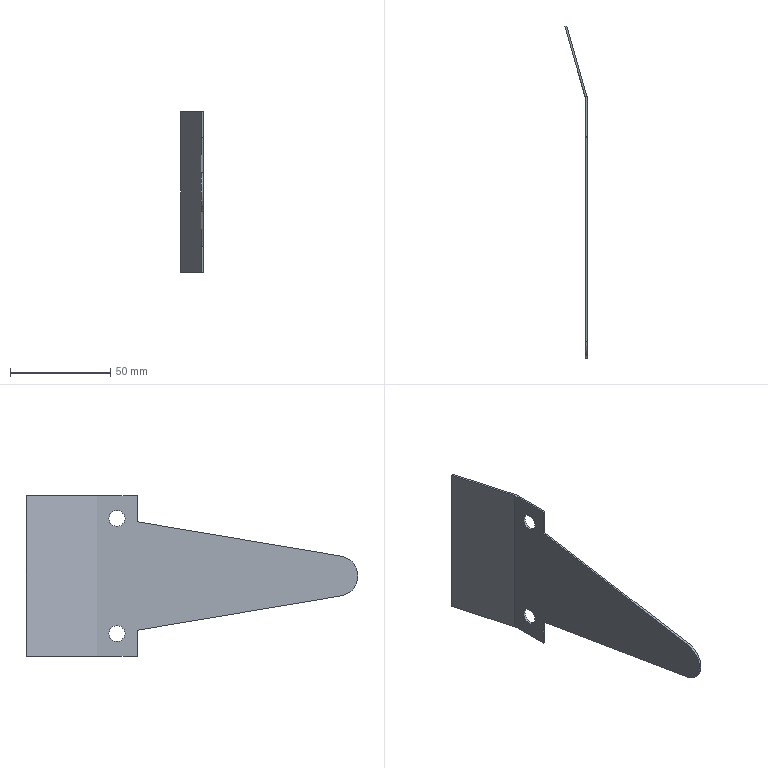Component | SolidWorks | OuterBagExpansionSheetMetal-1 | 2 solids | 21 faces | box 11.04 x 165.28 x 80 mm | volume 8295 mm3 | plane 15 | cylinder 6 | commonest cylinder face diameters 8 x4 2 x1 20 x1
build123d program:
from build123d import *

# Parameters (mm, degrees)
BOSS_EXTRUDE1_DEPTH = 1
SKETCH3_R           = 4
CUT_EXTRUDE1_DEPTH  = 10
BOSS_EXTRUDE2_DEPTH = 80


with BuildPart() as part:
    # Sketch2 → Boss-Extrude1 (new body)
    with BuildSketch(Plane.XY):
        with BuildLine():
            Line((0.831, 140.622), (102.493, 157.762))
            ThreePointArc((102.493, 157.762), (110.831, 167.622), (102.493, 177.483))
            Line((102.493, 177.483), (0.831, 194.622))
            Line((0.831, 194.622), (0.831, 207.622))
            Line((0.831, 207.622), (-19.169, 207.622))
            Line((-19.169, 207.622), (-19.169, 127.622))
            Line((-19.169, 127.622), (0.831, 127.622))
            Line((0.831, 127.622), (0.831, 140.622))
        make_face()
    extrude(amount=BOSS_EXTRUDE1_DEPTH)

    # Sketch3 → Cut-Extrude1 (cut)
    with BuildSketch(Plane.XY.offset(1)):
        with Locations((-9.169, 138.937)):
            Circle(SKETCH3_R)
        with Locations((-9.169, 196.308)):
            Circle(SKETCH3_R)
    extrude(amount=-CUT_EXTRUDE1_DEPTH, mode=Mode.SUBTRACT)


with BuildPart() as body_2:
    # Sketch4 → Boss-Extrude2 (new body)
    with BuildSketch(Plane(origin=(0, 207.622, 0), x_dir=(1, 0, 0), z_dir=(0, 1, 0))):
        with BuildLine():
            Line((-19.169, -1), (-19.169, 0))
            Line((-19.169, 0), (-54.169, 10.036))
            Line((-54.169, 10.036), (-54.445, 9.075))
            Line((-54.445, 9.075), (-19.445, -0.9613))
            ThreePointArc((-19.445, -0.9613), (-19.308, -0.9903), (-19.169, -1))
        make_face()
    extrude(amount=-BOSS_EXTRUDE2_DEPTH)


solid = Compound([part.part, body_2.part])

# Placed as in the assembly
solid = solid.moved(Location((-550.446, 3.257, 541.09), (-90, 90, 0)))
STEP:
#1=COLOUR_RGB('',0.7922,0.8196,0.9333);
#2=FILL_AREA_STYLE_COLOUR('',#1);
#3=FILL_AREA_STYLE('',(#2));
#4=SURFACE_STYLE_FILL_AREA(#3);
#5=SURFACE_SIDE_STYLE('',(#4));
#6=SURFACE_STYLE_USAGE(.BOTH.,#5);
#7=PRESENTATION_STYLE_ASSIGNMENT((#6));
#8=CARTESIAN_POINT('',(-21.633,0.8938,13.129));
#9=VERTEX_POINT('',#8);
#10=CARTESIAN_POINT('',(-21.632,0.8829,13.129));
#11=VERTEX_POINT('',#10);
#12=CARTESIAN_POINT('',(-21.671,0.8829,13.129));
#13=DIRECTION('',(0.,0.,-1.));
#14=DIRECTION('',(1.,0.,0.));
#15=AXIS2_PLACEMENT_3D('',#12,#13,#14);
#16=CIRCLE('',#15,0.03937);
#17=EDGE_CURVE('',#9,#11,#16,.T.);
#18=ORIENTED_EDGE('',*,*,#17,.F.);
#19=CARTESIAN_POINT('',(-21.633,0.8938,16.278));
#20=VERTEX_POINT('',#19);
#21=CARTESIAN_POINT('',(-21.633,0.8938,16.278));
#22=DIRECTION('',(0.,0.,-1.));
#23=VECTOR('',#22,39.37);
#24=LINE('',#21,#23);
#25=EDGE_CURVE('',#20,#9,#24,.T.);
#26=ORIENTED_EDGE('',*,*,#25,.F.);
#27=CARTESIAN_POINT('',(-21.632,0.8829,16.278));
#28=VERTEX_POINT('',#27);
#29=CARTESIAN_POINT('',(-21.671,0.8829,16.278));
#30=DIRECTION('',(0.,0.,-1.));
#31=DIRECTION('',(1.,0.,0.));
#32=AXIS2_PLACEMENT_3D('',#29,#30,#31);
#33=CIRCLE('',#32,0.03937);
#34=EDGE_CURVE('',#20,#28,#33,.T.);
#35=ORIENTED_EDGE('',*,*,#34,.T.);
#36=CARTESIAN_POINT('',(-21.632,0.8829,16.278));
#37=DIRECTION('',(0.,0.,-1.));
#38=VECTOR('',#37,39.37);
#39=LINE('',#36,#38);
#40=EDGE_CURVE('',#28,#11,#39,.T.);
#41=ORIENTED_EDGE('',*,*,#40,.T.);
#42=EDGE_LOOP('',(#18,#26,#35,#41));
#43=FACE_OUTER_BOUND('',#42,.T.);
#44=CARTESIAN_POINT('',(-21.671,0.8829,16.278));
#45=DIRECTION('',(0.,0.,-1.));
#46=DIRECTION('',(1.,0.,0.));
#47=AXIS2_PLACEMENT_3D('',#44,#45,#46);
#48=CYLINDRICAL_SURFACE('',#47,0.03937);
#49=ADVANCED_FACE('',(#43),#48,.T.);
#50=CARTESIAN_POINT('',(-22.028,2.272,13.129));
#51=VERTEX_POINT('',#50);
#52=CARTESIAN_POINT('',(-21.633,0.8938,13.129));
#53=DIRECTION('',(0.2756,-0.9613,-0.));
#54=VECTOR('',#53,39.37);
#55=LINE('',#52,#54);
#56=EDGE_CURVE('',#51,#9,#55,.T.);
#57=ORIENTED_EDGE('',*,*,#56,.F.);
#58=CARTESIAN_POINT('',(-22.028,2.272,16.278));
#59=VERTEX_POINT('',#58);
#60=CARTESIAN_POINT('',(-22.028,2.272,16.278));
#61=DIRECTION('',(0.,0.,-1.));
#62=VECTOR('',#61,39.37);
#63=LINE('',#60,#62);
#64=EDGE_CURVE('',#59,#51,#63,.T.);
#65=ORIENTED_EDGE('',*,*,#64,.F.);
#66=CARTESIAN_POINT('',(-21.633,0.8938,16.278));
#67=DIRECTION('',(0.2756,-0.9613,-0.));
#68=VECTOR('',#67,39.37);
#69=LINE('',#66,#68);
#70=EDGE_CURVE('',#59,#20,#69,.T.);
#71=ORIENTED_EDGE('',*,*,#70,.T.);
#72=ORIENTED_EDGE('',*,*,#25,.T.);
#73=EDGE_LOOP('',(#57,#65,#71,#72));
#74=FACE_OUTER_BOUND('',#73,.T.);
#75=CARTESIAN_POINT('',(-21.633,0.8938,16.278));
#76=DIRECTION('',(0.9613,0.2756,0.));
#77=DIRECTION('',(0.2756,-0.9613,-0.));
#78=AXIS2_PLACEMENT_3D('',#75,#76,#77);
#79=PLANE('',#78);
#80=ADVANCED_FACE('',(#74),#79,.T.);
#81=CARTESIAN_POINT('',(-22.066,2.261,13.129));
#82=VERTEX_POINT('',#81);
#83=CARTESIAN_POINT('',(-22.066,2.261,13.129));
#84=DIRECTION('',(0.9613,0.2756,0.));
#85=VECTOR('',#84,39.37);
#86=LINE('',#83,#85);
#87=EDGE_CURVE('',#82,#51,#86,.T.);
#88=ORIENTED_EDGE('',*,*,#87,.F.);
#89=CARTESIAN_POINT('',(-22.066,2.261,16.278));
#90=VERTEX_POINT('',#89);
#91=CARTESIAN_POINT('',(-22.066,2.261,16.278));
#92=DIRECTION('',(0.,0.,-1.));
#93=VECTOR('',#92,39.37);
#94=LINE('',#91,#93);
#95=EDGE_CURVE('',#90,#82,#94,.T.);
#96=ORIENTED_EDGE('',*,*,#95,.F.);
#97=CARTESIAN_POINT('',(-22.066,2.261,16.278));
#98=DIRECTION('',(0.9613,0.2756,0.));
#99=VECTOR('',#98,39.37);
#100=LINE('',#97,#99);
#101=EDGE_CURVE('',#90,#59,#100,.T.);
#102=ORIENTED_EDGE('',*,*,#101,.T.);
#103=ORIENTED_EDGE('',*,*,#64,.T.);
#104=EDGE_LOOP('',(#88,#96,#102,#103));
#105=FACE_OUTER_BOUND('',#104,.T.);
#106=CARTESIAN_POINT('',(-22.066,2.261,16.278));
#107=DIRECTION('',(-0.2756,0.9613,0.));
#108=DIRECTION('',(0.9613,0.2756,0.));
#109=AXIS2_PLACEMENT_3D('',#106,#107,#108);
#110=PLANE('',#109);
#111=ADVANCED_FACE('',(#105),#110,.T.);
#112=CARTESIAN_POINT('',(-21.671,0.8829,13.129));
#113=VERTEX_POINT('',#112);
#114=CARTESIAN_POINT('',(-21.671,0.8829,13.129));
#115=DIRECTION('',(-0.2756,0.9613,0.));
#116=VECTOR('',#115,39.37);
#117=LINE('',#114,#116);
#118=EDGE_CURVE('',#113,#82,#117,.T.);
#119=ORIENTED_EDGE('',*,*,#118,.F.);
#120=CARTESIAN_POINT('',(-21.671,0.8829,16.278));
#121=VERTEX_POINT('',#120);
#122=CARTESIAN_POINT('',(-21.671,0.8829,16.278));
#123=DIRECTION('',(0.,0.,-1.));
#124=VECTOR('',#123,39.37);
#125=LINE('',#122,#124);
#126=EDGE_CURVE('',#121,#113,#125,.T.);
#127=ORIENTED_EDGE('',*,*,#126,.F.);
#128=CARTESIAN_POINT('',(-21.671,0.8829,16.278));
#129=DIRECTION('',(-0.2756,0.9613,0.));
#130=VECTOR('',#129,39.37);
#131=LINE('',#128,#130);
#132=EDGE_CURVE('',#121,#90,#131,.T.);
#133=ORIENTED_EDGE('',*,*,#132,.T.);
#134=ORIENTED_EDGE('',*,*,#95,.T.);
#135=EDGE_LOOP('',(#119,#127,#133,#134));
#136=FACE_OUTER_BOUND('',#135,.T.);
#137=CARTESIAN_POINT('',(-21.671,0.8829,16.278));
#138=DIRECTION('',(-0.9613,-0.2756,-0.));
#139=DIRECTION('',(-0.2756,0.9613,0.));
#140=AXIS2_PLACEMENT_3D('',#137,#138,#139);
#141=PLANE('',#140);
#142=ADVANCED_FACE('',(#136),#141,.T.);
#143=CARTESIAN_POINT('',(-21.632,0.8829,13.129));
#144=DIRECTION('',(-1.,0.,-0.));
#145=VECTOR('',#144,39.37);
#146=LINE('',#143,#145);
#147=EDGE_CURVE('',#11,#113,#146,.T.);
#148=ORIENTED_EDGE('',*,*,#147,.F.);
#149=ORIENTED_EDGE('',*,*,#40,.F.);
#150=CARTESIAN_POINT('',(-21.632,0.8829,16.278));
#151=DIRECTION('',(-1.,0.,-0.));
#152=VECTOR('',#151,39.37);
#153=LINE('',#150,#152);
#154=EDGE_CURVE('',#28,#121,#153,.T.);
#155=ORIENTED_EDGE('',*,*,#154,.T.);
#156=ORIENTED_EDGE('',*,*,#126,.T.);
#157=EDGE_LOOP('',(#148,#149,#155,#156));
#158=FACE_OUTER_BOUND('',#157,.T.);
#159=CARTESIAN_POINT('',(-21.632,0.8829,16.278));
#160=DIRECTION('',(-0.,-1.,-0.));
#161=DIRECTION('',(-1.,0.,-0.));
#162=AXIS2_PLACEMENT_3D('',#159,#160,#161);
#163=PLANE('',#162);
#164=ADVANCED_FACE('',(#158),#163,.T.);
#165=ORIENTED_EDGE('',*,*,#34,.F.);
#166=ORIENTED_EDGE('',*,*,#70,.F.);
#167=ORIENTED_EDGE('',*,*,#101,.F.);
#168=ORIENTED_EDGE('',*,*,#132,.F.);
#169=ORIENTED_EDGE('',*,*,#154,.F.);
#170=EDGE_LOOP('',(#165,#166,#167,#168,#169));
#171=FACE_OUTER_BOUND('',#170,.T.);
#172=CARTESIAN_POINT('',(-21.671,0.8829,16.278));
#173=DIRECTION('',(0.,0.,-1.));
#174=DIRECTION('',(1.,-0.,0.));
#175=AXIS2_PLACEMENT_3D('',#172,#173,#174);
#176=PLANE('',#175);
#177=ADVANCED_FACE('',(#171),#176,.F.);
#178=ORIENTED_EDGE('',*,*,#17,.T.);
#179=ORIENTED_EDGE('',*,*,#147,.T.);
#180=ORIENTED_EDGE('',*,*,#118,.T.);
#181=ORIENTED_EDGE('',*,*,#87,.T.);
#182=ORIENTED_EDGE('',*,*,#56,.T.);
#183=EDGE_LOOP('',(#178,#179,#180,#181,#182));
#184=FACE_OUTER_BOUND('',#183,.T.);
#185=CARTESIAN_POINT('',(-21.671,0.8829,13.129));
#186=DIRECTION('',(0.,0.,-1.));
#187=DIRECTION('',(1.,-0.,0.));
#188=AXIS2_PLACEMENT_3D('',#185,#186,#187);
#189=PLANE('',#188);
#190=ADVANCED_FACE('',(#184),#189,.T.);
#191=CLOSED_SHELL('',(#49,#80,#111,#142,#164,#177,#190));
#192=MANIFOLD_SOLID_BREP('',#191);
#193=STYLED_ITEM('',(#7),#192);
#194=PRESENTATION_LAYER_ASSIGNMENT('','',(#193));
#195=(LENGTH_UNIT()NAMED_UNIT(*)SI_UNIT($,.METRE.));
#196=LENGTH_MEASURE_WITH_UNIT(LENGTH_MEASURE(0.0254),#195);
#197=DIMENSIONAL_EXPONENTS(1.,0.,0.,0.,0.,0.,0.);
#198=(CONVERSION_BASED_UNIT('',#196)LENGTH_UNIT()NAMED_UNIT(#197));
#199=UNCERTAINTY_MEASURE_WITH_UNIT(LENGTH_MEASURE(0.00001),#198,'','');
#200=(NAMED_UNIT(*)PLANE_ANGLE_UNIT()SI_UNIT($,.RADIAN.));
#201=(NAMED_UNIT(*)SI_UNIT($,.STERADIAN.)SOLID_ANGLE_UNIT());
#202=(GEOMETRIC_REPRESENTATION_CONTEXT(3)GLOBAL_UNCERTAINTY_ASSIGNED_CONTEXT((#199))GLOBAL_UNIT_ASSIGNED_CONTEXT((#198,#200,#201))REPRESENTATION_CONTEXT('',''));
#203=MECHANICAL_DESIGN_GEOMETRIC_PRESENTATION_REPRESENTATION('',(#193),#202);
#204=COLOUR_RGB('',0.7922,0.8196,0.9333);
#205=FILL_AREA_STYLE_COLOUR('',#204);
#206=FILL_AREA_STYLE('',(#205));
#207=SURFACE_STYLE_FILL_AREA(#206);
#208=SURFACE_SIDE_STYLE('',(#207));
#209=SURFACE_STYLE_USAGE(.BOTH.,#208);
#210=PRESENTATION_STYLE_ASSIGNMENT((#209));
#211=CARTESIAN_POINT('',(-21.671,0.6467,15.833));
#212=VERTEX_POINT('',#211);
#213=CARTESIAN_POINT('',(-21.671,0.3317,15.833));
#214=VERTEX_POINT('',#213);
#215=CARTESIAN_POINT('',(-21.671,0.4892,15.833));
#216=DIRECTION('',(1.,-0.,0.));
#217=DIRECTION('',(0.,-1.,0.));
#218=AXIS2_PLACEMENT_3D('',#215,#216,#217);
#219=CIRCLE('',#218,0.1575);
#220=EDGE_CURVE('',#212,#214,#219,.T.);
#221=ORIENTED_EDGE('',*,*,#220,.F.);
#222=CARTESIAN_POINT('',(-21.632,0.6467,15.833));
#223=VERTEX_POINT('',#222);
#224=CARTESIAN_POINT('',(-22.025,0.6467,15.833));
#225=DIRECTION('',(1.,-0.,0.));
#226=VECTOR('',#225,39.37);
#227=LINE('',#224,#226);
#228=EDGE_CURVE('',#212,#223,#227,.T.);
#229=ORIENTED_EDGE('',*,*,#228,.T.);
#230=CARTESIAN_POINT('',(-21.632,0.3317,15.833));
#231=VERTEX_POINT('',#230);
#232=CARTESIAN_POINT('',(-21.632,0.4892,15.833));
#233=DIRECTION('',(1.,-0.,0.));
#234=DIRECTION('',(0.,-1.,0.));
#235=AXIS2_PLACEMENT_3D('',#232,#233,#234);
#236=CIRCLE('',#235,0.1575);
#237=EDGE_CURVE('',#223,#231,#236,.T.);
#238=ORIENTED_EDGE('',*,*,#237,.T.);
#239=CARTESIAN_POINT('',(-22.025,0.3317,15.833));
#240=DIRECTION('',(1.,-0.,0.));
#241=VECTOR('',#240,39.37);
#242=LINE('',#239,#241);
#243=EDGE_CURVE('',#214,#231,#242,.T.);
#244=ORIENTED_EDGE('',*,*,#243,.F.);
#245=EDGE_LOOP('',(#221,#229,#238,#244));
#246=FACE_OUTER_BOUND('',#245,.T.);
#247=CARTESIAN_POINT('',(-22.025,0.4892,15.833));
#248=DIRECTION('',(1.,-0.,0.));
#249=DIRECTION('',(0.,-1.,0.));
#250=AXIS2_PLACEMENT_3D('',#247,#248,#249);
#251=CYLINDRICAL_SURFACE('',#250,0.1575);
#252=ADVANCED_FACE('',(#246),#251,.F.);
#253=CARTESIAN_POINT('',(-21.671,0.6467,13.574));
#254=VERTEX_POINT('',#253);
#255=CARTESIAN_POINT('',(-21.671,0.3317,13.574));
#256=VERTEX_POINT('',#255);
#257=CARTESIAN_POINT('',(-21.671,0.4892,13.574));
#258=DIRECTION('',(1.,-0.,0.));
#259=DIRECTION('',(0.,-1.,0.));
#260=AXIS2_PLACEMENT_3D('',#257,#258,#259);
#261=CIRCLE('',#260,0.1575);
#262=EDGE_CURVE('',#254,#256,#261,.T.);
#263=ORIENTED_EDGE('',*,*,#262,.F.);
#264=CARTESIAN_POINT('',(-21.632,0.6467,13.574));
#265=VERTEX_POINT('',#264);
#266=CARTESIAN_POINT('',(-22.025,0.6467,13.574));
#267=DIRECTION('',(1.,-0.,0.));
#268=VECTOR('',#267,39.37);
#269=LINE('',#266,#268);
#270=EDGE_CURVE('',#254,#265,#269,.T.);
#271=ORIENTED_EDGE('',*,*,#270,.T.);
#272=CARTESIAN_POINT('',(-21.632,0.3317,13.574));
#273=VERTEX_POINT('',#272);
#274=CARTESIAN_POINT('',(-21.632,0.4892,13.574));
#275=DIRECTION('',(1.,-0.,0.));
#276=DIRECTION('',(0.,1.,0.));
#277=AXIS2_PLACEMENT_3D('',#274,#275,#276);
#278=CIRCLE('',#277,0.1575);
#279=EDGE_CURVE('',#265,#273,#278,.T.);
#280=ORIENTED_EDGE('',*,*,#279,.T.);
#281=CARTESIAN_POINT('',(-22.025,0.3317,13.574));
#282=DIRECTION('',(1.,-0.,0.));
#283=VECTOR('',#282,39.37);
#284=LINE('',#281,#283);
#285=EDGE_CURVE('',#256,#273,#284,.T.);
#286=ORIENTED_EDGE('',*,*,#285,.F.);
#287=EDGE_LOOP('',(#263,#271,#280,#286));
#288=FACE_OUTER_BOUND('',#287,.T.);
#289=CARTESIAN_POINT('',(-22.025,0.4892,13.574));
#290=DIRECTION('',(1.,-0.,0.));
#291=DIRECTION('',(0.,-1.,0.));
#292=AXIS2_PLACEMENT_3D('',#289,#290,#291);
#293=CYLINDRICAL_SURFACE('',#292,0.1575);
#294=ADVANCED_FACE('',(#288),#293,.F.);
#295=CARTESIAN_POINT('',(-21.671,-3.907,15.092));
#296=VERTEX_POINT('',#295);
#297=CARTESIAN_POINT('',(-21.671,-3.907,14.315));
#298=VERTEX_POINT('',#297);
#299=CARTESIAN_POINT('',(-21.671,-3.841,14.703));
#300=DIRECTION('',(1.,-0.,0.));
#301=DIRECTION('',(0.,-1.,0.));
#302=AXIS2_PLACEMENT_3D('',#299,#300,#301);
#303=CIRCLE('',#302,0.3937);
#304=EDGE_CURVE('',#296,#298,#303,.T.);
#305=ORIENTED_EDGE('',*,*,#304,.T.);
#306=CARTESIAN_POINT('',(-21.632,-3.907,14.315));
#307=VERTEX_POINT('',#306);
#308=CARTESIAN_POINT('',(-21.632,-3.907,14.315));
#309=DIRECTION('',(-1.,0.,-0.));
#310=VECTOR('',#309,39.37);
#311=LINE('',#308,#310);
#312=EDGE_CURVE('',#307,#298,#311,.T.);
#313=ORIENTED_EDGE('',*,*,#312,.F.);
#314=CARTESIAN_POINT('',(-21.632,-3.907,15.092));
#315=VERTEX_POINT('',#314);
#316=CARTESIAN_POINT('',(-21.632,-3.841,14.703));
#317=DIRECTION('',(1.,-0.,0.));
#318=DIRECTION('',(0.,-1.,0.));
#319=AXIS2_PLACEMENT_3D('',#316,#317,#318);
#320=CIRCLE('',#319,0.3937);
#321=EDGE_CURVE('',#315,#307,#320,.T.);
#322=ORIENTED_EDGE('',*,*,#321,.F.);
#323=CARTESIAN_POINT('',(-21.632,-3.907,15.092));
#324=DIRECTION('',(-1.,0.,-0.));
#325=VECTOR('',#324,39.37);
#326=LINE('',#323,#325);
#327=EDGE_CURVE('',#315,#296,#326,.T.);
#328=ORIENTED_EDGE('',*,*,#327,.T.);
#329=EDGE_LOOP('',(#305,#313,#322,#328));
#330=FACE_OUTER_BOUND('',#329,.T.);
#331=CARTESIAN_POINT('',(-21.632,-3.841,14.703));
#332=DIRECTION('',(-1.,0.,-0.));
#333=DIRECTION('',(0.,1.,0.));
#334=AXIS2_PLACEMENT_3D('',#331,#332,#333);
#335=CYLINDRICAL_SURFACE('',#334,0.3937);
#336=ADVANCED_FACE('',(#330),#335,.T.);
#337=CARTESIAN_POINT('',(-21.671,0.09553,13.64));
#338=VERTEX_POINT('',#337);
#339=CARTESIAN_POINT('',(-21.671,-3.907,14.315));
#340=DIRECTION('',(0.,0.9861,-0.1662));
#341=VECTOR('',#340,39.37);
#342=LINE('',#339,#341);
#343=EDGE_CURVE('',#298,#338,#342,.T.);
#344=ORIENTED_EDGE('',*,*,#343,.T.);
#345=CARTESIAN_POINT('',(-21.632,0.09553,13.64));
#346=VERTEX_POINT('',#345);
#347=CARTESIAN_POINT('',(-21.632,0.09553,13.64));
#348=DIRECTION('',(-1.,0.,-0.));
#349=VECTOR('',#348,39.37);
#350=LINE('',#347,#349);
#351=EDGE_CURVE('',#346,#338,#350,.T.);
#352=ORIENTED_EDGE('',*,*,#351,.F.);
#353=CARTESIAN_POINT('',(-21.632,-3.907,14.315));
#354=DIRECTION('',(0.,0.9861,-0.1662));
#355=VECTOR('',#354,39.37);
#356=LINE('',#353,#355);
#357=EDGE_CURVE('',#307,#346,#356,.T.);
#358=ORIENTED_EDGE('',*,*,#357,.F.);
#359=ORIENTED_EDGE('',*,*,#312,.T.);
#360=EDGE_LOOP('',(#344,#352,#358,#359));
#361=FACE_OUTER_BOUND('',#360,.T.);
#362=CARTESIAN_POINT('',(-21.632,-3.907,14.315));
#363=DIRECTION('',(-0.,0.1662,0.9861));
#364=DIRECTION('',(-0.,-0.9861,0.1662));
#365=AXIS2_PLACEMENT_3D('',#362,#363,#364);
#366=PLANE('',#365);
#367=ADVANCED_FACE('',(#361),#366,.F.);
#368=CARTESIAN_POINT('',(-21.671,0.09553,13.129));
#369=VERTEX_POINT('',#368);
#370=CARTESIAN_POINT('',(-21.671,0.09553,13.64));
#371=DIRECTION('',(0.,0.,-1.));
#372=VECTOR('',#371,39.37);
#373=LINE('',#370,#372);
#374=EDGE_CURVE('',#338,#369,#373,.T.);
#375=ORIENTED_EDGE('',*,*,#374,.T.);
#376=CARTESIAN_POINT('',(-21.632,0.09553,13.129));
#377=VERTEX_POINT('',#376);
#378=CARTESIAN_POINT('',(-21.632,0.09553,13.129));
#379=DIRECTION('',(-1.,0.,-0.));
#380=VECTOR('',#379,39.37);
#381=LINE('',#378,#380);
#382=EDGE_CURVE('',#377,#369,#381,.T.);
#383=ORIENTED_EDGE('',*,*,#382,.F.);
#384=CARTESIAN_POINT('',(-21.632,0.09553,13.64));
#385=DIRECTION('',(0.,0.,-1.));
#386=VECTOR('',#385,39.37);
#387=LINE('',#384,#386);
#388=EDGE_CURVE('',#346,#377,#387,.T.);
#389=ORIENTED_EDGE('',*,*,#388,.F.);
#390=ORIENTED_EDGE('',*,*,#351,.T.);
#391=EDGE_LOOP('',(#375,#383,#389,#390));
#392=FACE_OUTER_BOUND('',#391,.T.);
#393=CARTESIAN_POINT('',(-21.632,0.09553,13.64));
#394=DIRECTION('',(0.,1.,0.));
#395=DIRECTION('',(1.,-0.,0.));
#396=AXIS2_PLACEMENT_3D('',#393,#394,#395);
#397=PLANE('',#396);
#398=ADVANCED_FACE('',(#392),#397,.F.);
#399=CARTESIAN_POINT('',(-21.671,0.8829,13.129));
#400=VERTEX_POINT('',#399);
#401=CARTESIAN_POINT('',(-21.671,0.8829,13.129));
#402=DIRECTION('',(0.,1.,0.));
#403=VECTOR('',#402,39.37);
#404=LINE('',#401,#403);
#405=EDGE_CURVE('',#369,#400,#404,.T.);
#406=ORIENTED_EDGE('',*,*,#405,.T.);
#407=CARTESIAN_POINT('',(-21.632,0.8829,13.129));
#408=VERTEX_POINT('',#407);
#409=CARTESIAN_POINT('',(-21.632,0.8829,13.129));
#410=DIRECTION('',(-1.,0.,-0.));
#411=VECTOR('',#410,39.37);
#412=LINE('',#409,#411);
#413=EDGE_CURVE('',#408,#400,#412,.T.);
#414=ORIENTED_EDGE('',*,*,#413,.F.);
#415=CARTESIAN_POINT('',(-21.632,0.8829,13.129));
#416=DIRECTION('',(0.,1.,0.));
#417=VECTOR('',#416,39.37);
#418=LINE('',#415,#417);
#419=EDGE_CURVE('',#377,#408,#418,.T.);
#420=ORIENTED_EDGE('',*,*,#419,.F.);
#421=ORIENTED_EDGE('',*,*,#382,.T.);
#422=EDGE_LOOP('',(#406,#414,#420,#421));
#423=FACE_OUTER_BOUND('',#422,.T.);
#424=CARTESIAN_POINT('',(-21.632,0.8829,13.129));
#425=DIRECTION('',(-0.,-0.,1.));
#426=DIRECTION('',(-1.,0.,-0.));
#427=AXIS2_PLACEMENT_3D('',#424,#425,#426);
#428=PLANE('',#427);
#429=ADVANCED_FACE('',(#423),#428,.F.);
#430=CARTESIAN_POINT('',(-21.671,0.8829,16.278));
#431=VERTEX_POINT('',#430);
#432=CARTESIAN_POINT('',(-21.671,0.8829,16.278));
#433=DIRECTION('',(-0.,-0.,1.));
#434=VECTOR('',#433,39.37);
#435=LINE('',#432,#434);
#436=EDGE_CURVE('',#400,#431,#435,.T.);
#437=ORIENTED_EDGE('',*,*,#436,.T.);
#438=CARTESIAN_POINT('',(-21.632,0.8829,16.278));
#439=VERTEX_POINT('',#438);
#440=CARTESIAN_POINT('',(-21.632,0.8829,16.278));
#441=DIRECTION('',(-1.,0.,-0.));
#442=VECTOR('',#441,39.37);
#443=LINE('',#440,#442);
#444=EDGE_CURVE('',#439,#431,#443,.T.);
#445=ORIENTED_EDGE('',*,*,#444,.F.);
#446=CARTESIAN_POINT('',(-21.632,0.8829,16.278));
#447=DIRECTION('',(-0.,-0.,1.));
#448=VECTOR('',#447,39.37);
#449=LINE('',#446,#448);
#450=EDGE_CURVE('',#408,#439,#449,.T.);
#451=ORIENTED_EDGE('',*,*,#450,.F.);
#452=ORIENTED_EDGE('',*,*,#413,.T.);
#453=EDGE_LOOP('',(#437,#445,#451,#452));
#454=FACE_OUTER_BOUND('',#453,.T.);
#455=CARTESIAN_POINT('',(-21.632,0.8829,16.278));
#456=DIRECTION('',(-0.,-1.,-0.));
#457=DIRECTION('',(-1.,0.,-0.));
#458=AXIS2_PLACEMENT_3D('',#455,#456,#457);
#459=PLANE('',#458);
#460=ADVANCED_FACE('',(#454),#459,.F.);
#461=CARTESIAN_POINT('',(-21.671,0.09553,16.278));
#462=VERTEX_POINT('',#461);
#463=CARTESIAN_POINT('',(-21.671,0.8829,16.278));
#464=DIRECTION('',(-0.,-1.,-0.));
#465=VECTOR('',#464,39.37);
#466=LINE('',#463,#465);
#467=EDGE_CURVE('',#431,#462,#466,.T.);
#468=ORIENTED_EDGE('',*,*,#467,.T.);
#469=CARTESIAN_POINT('',(-21.632,0.09553,16.278));
#470=VERTEX_POINT('',#469);
#471=CARTESIAN_POINT('',(-21.632,0.09553,16.278));
#472=DIRECTION('',(-1.,0.,-0.));
#473=VECTOR('',#472,39.37);
#474=LINE('',#471,#473);
#475=EDGE_CURVE('',#470,#462,#474,.T.);
#476=ORIENTED_EDGE('',*,*,#475,.F.);
#477=CARTESIAN_POINT('',(-21.632,0.8829,16.278));
#478=DIRECTION('',(-0.,-1.,-0.));
#479=VECTOR('',#478,39.37);
#480=LINE('',#477,#479);
#481=EDGE_CURVE('',#439,#470,#480,.T.);
#482=ORIENTED_EDGE('',*,*,#481,.F.);
#483=ORIENTED_EDGE('',*,*,#444,.T.);
#484=EDGE_LOOP('',(#468,#476,#482,#483));
#485=FACE_OUTER_BOUND('',#484,.T.);
#486=CARTESIAN_POINT('',(-21.632,0.8829,16.278));
#487=DIRECTION('',(0.,0.,-1.));
#488=DIRECTION('',(1.,-0.,0.));
#489=AXIS2_PLACEMENT_3D('',#486,#487,#488);
#490=PLANE('',#489);
#491=ADVANCED_FACE('',(#485),#490,.F.);
#492=CARTESIAN_POINT('',(-21.671,0.09553,15.766));
#493=VERTEX_POINT('',#492);
#494=CARTESIAN_POINT('',(-21.671,0.09553,16.278));
#495=DIRECTION('',(0.,0.,-1.));
#496=VECTOR('',#495,39.37);
#497=LINE('',#494,#496);
#498=EDGE_CURVE('',#462,#493,#497,.T.);
#499=ORIENTED_EDGE('',*,*,#498,.T.);
#500=CARTESIAN_POINT('',(-21.632,0.09553,15.766));
#501=VERTEX_POINT('',#500);
#502=CARTESIAN_POINT('',(-21.632,0.09553,15.766));
#503=DIRECTION('',(-1.,0.,-0.));
#504=VECTOR('',#503,39.37);
#505=LINE('',#502,#504);
#506=EDGE_CURVE('',#501,#493,#505,.T.);
#507=ORIENTED_EDGE('',*,*,#506,.F.);
#508=CARTESIAN_POINT('',(-21.632,0.09553,16.278));
#509=DIRECTION('',(0.,0.,-1.));
#510=VECTOR('',#509,39.37);
#511=LINE('',#508,#510);
#512=EDGE_CURVE('',#470,#501,#511,.T.);
#513=ORIENTED_EDGE('',*,*,#512,.F.);
#514=ORIENTED_EDGE('',*,*,#475,.T.);
#515=EDGE_LOOP('',(#499,#507,#513,#514));
#516=FACE_OUTER_BOUND('',#515,.T.);
#517=CARTESIAN_POINT('',(-21.632,0.09553,16.278));
#518=DIRECTION('',(0.,1.,0.));
#519=DIRECTION('',(1.,-0.,0.));
#520=AXIS2_PLACEMENT_3D('',#517,#518,#519);
#521=PLANE('',#520);
#522=ADVANCED_FACE('',(#516),#521,.F.);
#523=CARTESIAN_POINT('',(-21.671,0.09553,15.766));
#524=DIRECTION('',(0.,-0.9861,-0.1662));
#525=VECTOR('',#524,39.37);
#526=LINE('',#523,#525);
#527=EDGE_CURVE('',#493,#296,#526,.T.);
#528=ORIENTED_EDGE('',*,*,#527,.T.);
#529=ORIENTED_EDGE('',*,*,#327,.F.);
#530=CARTESIAN_POINT('',(-21.632,0.09553,15.766));
#531=DIRECTION('',(0.,-0.9861,-0.1662));
#532=VECTOR('',#531,39.37);
#533=LINE('',#530,#532);
#534=EDGE_CURVE('',#501,#315,#533,.T.);
#535=ORIENTED_EDGE('',*,*,#534,.F.);
#536=ORIENTED_EDGE('',*,*,#506,.T.);
#537=EDGE_LOOP('',(#528,#529,#535,#536));
#538=FACE_OUTER_BOUND('',#537,.T.);
#539=CARTESIAN_POINT('',(-21.632,0.09553,15.766));
#540=DIRECTION('',(0.,0.1662,-0.9861));
#541=DIRECTION('',(-0.,0.9861,0.1662));
#542=AXIS2_PLACEMENT_3D('',#539,#540,#541);
#543=PLANE('',#542);
#544=ADVANCED_FACE('',(#538),#543,.F.);
#545=CARTESIAN_POINT('',(-21.632,0.4892,15.833));
#546=DIRECTION('',(1.,-0.,0.));
#547=DIRECTION('',(0.,-1.,0.));
#548=AXIS2_PLACEMENT_3D('',#545,#546,#547);
#549=CIRCLE('',#548,0.1575);
#550=EDGE_CURVE('',#231,#223,#549,.T.);
#551=ORIENTED_EDGE('',*,*,#550,.F.);
#552=ORIENTED_EDGE('',*,*,#237,.F.);
#553=EDGE_LOOP('',(#551,#552));
#554=FACE_BOUND('',#553,.T.);
#555=CARTESIAN_POINT('',(-21.632,0.4892,13.574));
#556=DIRECTION('',(1.,-0.,0.));
#557=DIRECTION('',(0.,1.,0.));
#558=AXIS2_PLACEMENT_3D('',#555,#556,#557);
#559=CIRCLE('',#558,0.1575);
#560=EDGE_CURVE('',#273,#265,#559,.T.);
#561=ORIENTED_EDGE('',*,*,#560,.F.);
#562=ORIENTED_EDGE('',*,*,#279,.F.);
#563=EDGE_LOOP('',(#561,#562));
#564=FACE_BOUND('',#563,.T.);
#565=ORIENTED_EDGE('',*,*,#321,.T.);
#566=ORIENTED_EDGE('',*,*,#357,.T.);
#567=ORIENTED_EDGE('',*,*,#388,.T.);
#568=ORIENTED_EDGE('',*,*,#419,.T.);
#569=ORIENTED_EDGE('',*,*,#450,.T.);
#570=ORIENTED_EDGE('',*,*,#481,.T.);
#571=ORIENTED_EDGE('',*,*,#512,.T.);
#572=ORIENTED_EDGE('',*,*,#534,.T.);
#573=EDGE_LOOP('',(#565,#566,#567,#568,#569,#570,#571,#572));
#574=FACE_OUTER_BOUND('',#573,.T.);
#575=CARTESIAN_POINT('',(-21.632,-3.841,14.703));
#576=DIRECTION('',(1.,-0.,0.));
#577=DIRECTION('',(-0.,-1.,-0.));
#578=AXIS2_PLACEMENT_3D('',#575,#576,#577);
#579=PLANE('',#578);
#580=ADVANCED_FACE('',(#554,#564,#574),#579,.T.);
#581=CARTESIAN_POINT('',(-21.671,0.4892,15.833));
#582=DIRECTION('',(1.,-0.,0.));
#583=DIRECTION('',(0.,-1.,0.));
#584=AXIS2_PLACEMENT_3D('',#581,#582,#583);
#585=CIRCLE('',#584,0.1575);
#586=EDGE_CURVE('',#214,#212,#585,.T.);
#587=ORIENTED_EDGE('',*,*,#586,.T.);
#588=ORIENTED_EDGE('',*,*,#220,.T.);
#589=EDGE_LOOP('',(#587,#588));
#590=FACE_BOUND('',#589,.T.);
#591=CARTESIAN_POINT('',(-21.671,0.4892,13.574));
#592=DIRECTION('',(1.,-0.,0.));
#593=DIRECTION('',(0.,-1.,0.));
#594=AXIS2_PLACEMENT_3D('',#591,#592,#593);
#595=CIRCLE('',#594,0.1575);
#596=EDGE_CURVE('',#256,#254,#595,.T.);
#597=ORIENTED_EDGE('',*,*,#596,.T.);
#598=ORIENTED_EDGE('',*,*,#262,.T.);
#599=EDGE_LOOP('',(#597,#598));
#600=FACE_BOUND('',#599,.T.);
#601=ORIENTED_EDGE('',*,*,#304,.F.);
#602=ORIENTED_EDGE('',*,*,#527,.F.);
#603=ORIENTED_EDGE('',*,*,#498,.F.);
#604=ORIENTED_EDGE('',*,*,#467,.F.);
#605=ORIENTED_EDGE('',*,*,#436,.F.);
#606=ORIENTED_EDGE('',*,*,#405,.F.);
#607=ORIENTED_EDGE('',*,*,#374,.F.);
#608=ORIENTED_EDGE('',*,*,#343,.F.);
#609=EDGE_LOOP('',(#601,#602,#603,#604,#605,#606,#607,#608));
#610=FACE_OUTER_BOUND('',#609,.T.);
#611=CARTESIAN_POINT('',(-21.671,-3.841,14.703));
#612=DIRECTION('',(1.,-0.,0.));
#613=DIRECTION('',(-0.,-1.,-0.));
#614=AXIS2_PLACEMENT_3D('',#611,#612,#613);
#615=PLANE('',#614);
#616=ADVANCED_FACE('',(#590,#600,#610),#615,.F.);
#617=ORIENTED_EDGE('',*,*,#270,.F.);
#618=ORIENTED_EDGE('',*,*,#596,.F.);
#619=ORIENTED_EDGE('',*,*,#285,.T.);
#620=ORIENTED_EDGE('',*,*,#560,.T.);
#621=EDGE_LOOP('',(#617,#618,#619,#620));
#622=FACE_OUTER_BOUND('',#621,.T.);
#623=CARTESIAN_POINT('',(-22.025,0.4892,13.574));
#624=DIRECTION('',(1.,-0.,0.));
#625=DIRECTION('',(0.,-1.,0.));
#626=AXIS2_PLACEMENT_3D('',#623,#624,#625);
#627=CYLINDRICAL_SURFACE('',#626,0.1575);
#628=ADVANCED_FACE('',(#622),#627,.F.);
#629=ORIENTED_EDGE('',*,*,#228,.F.);
#630=ORIENTED_EDGE('',*,*,#586,.F.);
#631=ORIENTED_EDGE('',*,*,#243,.T.);
#632=ORIENTED_EDGE('',*,*,#550,.T.);
#633=EDGE_LOOP('',(#629,#630,#631,#632));
#634=FACE_OUTER_BOUND('',#633,.T.);
#635=CARTESIAN_POINT('',(-22.025,0.4892,15.833));
#636=DIRECTION('',(1.,-0.,0.));
#637=DIRECTION('',(0.,-1.,0.));
#638=AXIS2_PLACEMENT_3D('',#635,#636,#637);
#639=CYLINDRICAL_SURFACE('',#638,0.1575);
#640=ADVANCED_FACE('',(#634),#639,.F.);
#641=CLOSED_SHELL('',(#252,#294,#336,#367,#398,#429,#460,#491,#522,#544,#580,#616,#628,#640));
#642=MANIFOLD_SOLID_BREP('',#641);
#643=STYLED_ITEM('',(#210),#642);
#644=PRESENTATION_LAYER_ASSIGNMENT('','',(#643));
#645=CARTESIAN_POINT('',(0.,0.,0.));
#646=DIRECTION('',(0.,0.,1.));
#647=DIRECTION('',(1.,0.,0.));
#648=AXIS2_PLACEMENT_3D('',#645,#646,#647);
#649=(LENGTH_UNIT()NAMED_UNIT(*)SI_UNIT($,.METRE.));
#650=LENGTH_MEASURE_WITH_UNIT(LENGTH_MEASURE(0.0254),#649);
#651=DIMENSIONAL_EXPONENTS(1.,0.,0.,0.,0.,0.,0.);
#652=(CONVERSION_BASED_UNIT('',#650)LENGTH_UNIT()NAMED_UNIT(#651));
#653=UNCERTAINTY_MEASURE_WITH_UNIT(LENGTH_MEASURE(0.00001),#652,'','');
#654=(NAMED_UNIT(*)PLANE_ANGLE_UNIT()SI_UNIT($,.RADIAN.));
#655=(NAMED_UNIT(*)SI_UNIT($,.STERADIAN.)SOLID_ANGLE_UNIT());
#656=(GEOMETRIC_REPRESENTATION_CONTEXT(3)GLOBAL_UNCERTAINTY_ASSIGNED_CONTEXT((#653))GLOBAL_UNIT_ASSIGNED_CONTEXT((#652,#654,#655))REPRESENTATION_CONTEXT('',''));
#657=ADVANCED_BREP_SHAPE_REPRESENTATION('',(#192,#642,#648),#656);
#658=(LENGTH_UNIT()NAMED_UNIT(*)SI_UNIT($,.METRE.));
#659=LENGTH_MEASURE_WITH_UNIT(LENGTH_MEASURE(0.0254),#658);
#660=DIMENSIONAL_EXPONENTS(1.,0.,0.,0.,0.,0.,0.);
#661=(CONVERSION_BASED_UNIT('',#659)LENGTH_UNIT()NAMED_UNIT(#660));
#662=UNCERTAINTY_MEASURE_WITH_UNIT(LENGTH_MEASURE(0.00001),#661,'','');
#663=(NAMED_UNIT(*)PLANE_ANGLE_UNIT()SI_UNIT($,.RADIAN.));
#664=(NAMED_UNIT(*)SI_UNIT($,.STERADIAN.)SOLID_ANGLE_UNIT());
#665=(GEOMETRIC_REPRESENTATION_CONTEXT(3)GLOBAL_UNCERTAINTY_ASSIGNED_CONTEXT((#662))GLOBAL_UNIT_ASSIGNED_CONTEXT((#661,#663,#664))REPRESENTATION_CONTEXT('',''));
#666=MECHANICAL_DESIGN_GEOMETRIC_PRESENTATION_REPRESENTATION('',(#643),#665);